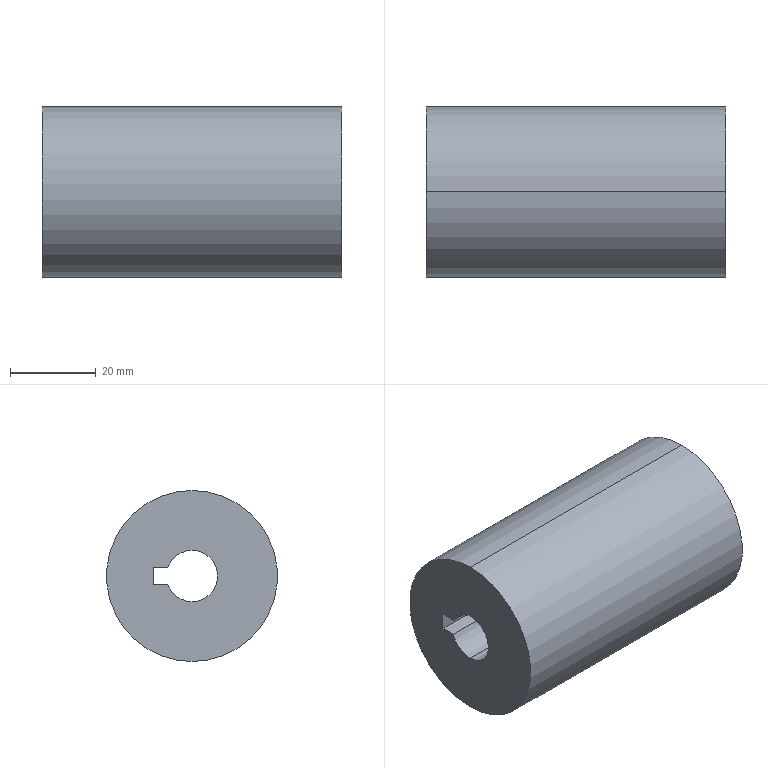Component | SolidWorks | Coupling2-1 | 1 solid | 10 faces | box 70 x 40 x 40 mm | volume 79176 mm3 | cylinder 5 | plane 5 | commonest cylinder face diameters 12 x3 40 x2
build123d program:
from build123d import *

# Parameters (mm, degrees)
SKETCH1_R      = 20
EXTRUDE1_DEPTH = 70


with BuildPart() as part:
    # Sketch1 → Extrude1 (new body)
    with BuildSketch(Plane.XY):
        Circle(SKETCH1_R)
        with BuildLine():
            Line((-2, 9), (2, 9))
            Line((2, 9), (2, 5.657))
            ThreePointArc((2, 5.657), (0, -6), (-2, 5.657))
            Line((-2, 5.657), (-2, 9))
        make_face(mode=Mode.SUBTRACT)
    extrude(amount=EXTRUDE1_DEPTH)


solid = part.part

# Placed as in the assembly
solid = solid.moved(Location((-87.284, 175.983, 58.736), (0, 90, 0)))
STEP:
#1=CARTESIAN_POINT('',(-0.6805,6.928,2.549));
#2=VERTEX_POINT('',#1);
#3=CARTESIAN_POINT('',(-0.6805,6.928,2.076));
#4=VERTEX_POINT('',#3);
#5=CARTESIAN_POINT('',(-0.6805,6.928,2.312));
#6=DIRECTION('',(1.,0.,0.));
#7=DIRECTION('',(0.,0.,-1.));
#8=AXIS2_PLACEMENT_3D('',#5,#6,#7);
#9=CIRCLE('',#8,0.2362);
#10=EDGE_CURVE('',#2,#4,#9,.T.);
#11=ORIENTED_EDGE('',*,*,#10,.T.);
#12=CARTESIAN_POINT('',(-3.436,6.928,2.076));
#13=VERTEX_POINT('',#12);
#14=CARTESIAN_POINT('',(-0.6805,6.928,2.076));
#15=DIRECTION('',(-1.,-0.,-0.));
#16=VECTOR('',#15,39.37);
#17=LINE('',#14,#16);
#18=EDGE_CURVE('',#4,#13,#17,.T.);
#19=ORIENTED_EDGE('',*,*,#18,.T.);
#20=CARTESIAN_POINT('',(-3.436,6.928,2.549));
#21=VERTEX_POINT('',#20);
#22=CARTESIAN_POINT('',(-3.436,6.928,2.312));
#23=DIRECTION('',(1.,0.,0.));
#24=DIRECTION('',(0.,0.,-1.));
#25=AXIS2_PLACEMENT_3D('',#22,#23,#24);
#26=CIRCLE('',#25,0.2362);
#27=EDGE_CURVE('',#21,#13,#26,.T.);
#28=ORIENTED_EDGE('',*,*,#27,.F.);
#29=CARTESIAN_POINT('',(-0.6805,6.928,2.549));
#30=DIRECTION('',(-1.,-0.,-0.));
#31=VECTOR('',#30,39.37);
#32=LINE('',#29,#31);
#33=EDGE_CURVE('',#2,#21,#32,.T.);
#34=ORIENTED_EDGE('',*,*,#33,.F.);
#35=EDGE_LOOP('',(#11,#19,#28,#34));
#36=FACE_OUTER_BOUND('',#35,.T.);
#37=CARTESIAN_POINT('',(-0.6805,6.928,2.312));
#38=DIRECTION('',(-1.,-0.,-0.));
#39=DIRECTION('',(0.,0.,1.));
#40=AXIS2_PLACEMENT_3D('',#37,#38,#39);
#41=CYLINDRICAL_SURFACE('',#40,0.2362);
#42=ADVANCED_FACE('',(#36),#41,.F.);
#43=CARTESIAN_POINT('',(-0.6805,7.151,2.391));
#44=VERTEX_POINT('',#43);
#45=CARTESIAN_POINT('',(-0.6805,6.928,2.312));
#46=DIRECTION('',(1.,0.,0.));
#47=DIRECTION('',(0.,0.,-1.));
#48=AXIS2_PLACEMENT_3D('',#45,#46,#47);
#49=CIRCLE('',#48,0.2362);
#50=EDGE_CURVE('',#44,#2,#49,.T.);
#51=ORIENTED_EDGE('',*,*,#50,.T.);
#52=ORIENTED_EDGE('',*,*,#33,.T.);
#53=CARTESIAN_POINT('',(-3.436,7.151,2.391));
#54=VERTEX_POINT('',#53);
#55=CARTESIAN_POINT('',(-3.436,6.928,2.312));
#56=DIRECTION('',(1.,0.,0.));
#57=DIRECTION('',(0.,0.,-1.));
#58=AXIS2_PLACEMENT_3D('',#55,#56,#57);
#59=CIRCLE('',#58,0.2362);
#60=EDGE_CURVE('',#54,#21,#59,.T.);
#61=ORIENTED_EDGE('',*,*,#60,.F.);
#62=CARTESIAN_POINT('',(-0.6805,7.151,2.391));
#63=DIRECTION('',(-1.,-0.,-0.));
#64=VECTOR('',#63,39.37);
#65=LINE('',#62,#64);
#66=EDGE_CURVE('',#44,#54,#65,.T.);
#67=ORIENTED_EDGE('',*,*,#66,.F.);
#68=EDGE_LOOP('',(#51,#52,#61,#67));
#69=FACE_OUTER_BOUND('',#68,.T.);
#70=CARTESIAN_POINT('',(-0.6805,6.928,2.312));
#71=DIRECTION('',(-1.,-0.,-0.));
#72=DIRECTION('',(0.,0.,1.));
#73=AXIS2_PLACEMENT_3D('',#70,#71,#72);
#74=CYLINDRICAL_SURFACE('',#73,0.2362);
#75=ADVANCED_FACE('',(#69),#74,.F.);
#76=CARTESIAN_POINT('',(-0.6805,6.928,1.525));
#77=VERTEX_POINT('',#76);
#78=CARTESIAN_POINT('',(-0.6805,6.928,3.1));
#79=VERTEX_POINT('',#78);
#80=CARTESIAN_POINT('',(-0.6805,6.928,2.312));
#81=DIRECTION('',(1.,0.,0.));
#82=DIRECTION('',(0.,0.,-1.));
#83=AXIS2_PLACEMENT_3D('',#80,#81,#82);
#84=CIRCLE('',#83,0.7874);
#85=EDGE_CURVE('',#77,#79,#84,.T.);
#86=ORIENTED_EDGE('',*,*,#85,.F.);
#87=CARTESIAN_POINT('',(-3.436,6.928,1.525));
#88=VERTEX_POINT('',#87);
#89=CARTESIAN_POINT('',(-0.6805,6.928,1.525));
#90=DIRECTION('',(-1.,-0.,-0.));
#91=VECTOR('',#90,39.37);
#92=LINE('',#89,#91);
#93=EDGE_CURVE('',#77,#88,#92,.T.);
#94=ORIENTED_EDGE('',*,*,#93,.T.);
#95=CARTESIAN_POINT('',(-3.436,6.928,3.1));
#96=VERTEX_POINT('',#95);
#97=CARTESIAN_POINT('',(-3.436,6.928,2.312));
#98=DIRECTION('',(1.,0.,0.));
#99=DIRECTION('',(0.,0.,-1.));
#100=AXIS2_PLACEMENT_3D('',#97,#98,#99);
#101=CIRCLE('',#100,0.7874);
#102=EDGE_CURVE('',#88,#96,#101,.T.);
#103=ORIENTED_EDGE('',*,*,#102,.T.);
#104=CARTESIAN_POINT('',(-0.6805,6.928,3.1));
#105=DIRECTION('',(-1.,-0.,-0.));
#106=VECTOR('',#105,39.37);
#107=LINE('',#104,#106);
#108=EDGE_CURVE('',#79,#96,#107,.T.);
#109=ORIENTED_EDGE('',*,*,#108,.F.);
#110=EDGE_LOOP('',(#86,#94,#103,#109));
#111=FACE_OUTER_BOUND('',#110,.T.);
#112=CARTESIAN_POINT('',(-0.6805,6.928,2.312));
#113=DIRECTION('',(-1.,-0.,-0.));
#114=DIRECTION('',(0.,0.,1.));
#115=AXIS2_PLACEMENT_3D('',#112,#113,#114);
#116=CYLINDRICAL_SURFACE('',#115,0.7874);
#117=ADVANCED_FACE('',(#111),#116,.T.);
#118=CARTESIAN_POINT('',(-0.6805,6.928,2.312));
#119=DIRECTION('',(1.,0.,0.));
#120=DIRECTION('',(0.,0.,-1.));
#121=AXIS2_PLACEMENT_3D('',#118,#119,#120);
#122=CIRCLE('',#121,0.7874);
#123=EDGE_CURVE('',#79,#77,#122,.T.);
#124=ORIENTED_EDGE('',*,*,#123,.T.);
#125=ORIENTED_EDGE('',*,*,#85,.T.);
#126=EDGE_LOOP('',(#124,#125));
#127=FACE_OUTER_BOUND('',#126,.T.);
#128=ORIENTED_EDGE('',*,*,#50,.F.);
#129=CARTESIAN_POINT('',(-0.6805,7.283,2.391));
#130=VERTEX_POINT('',#129);
#131=CARTESIAN_POINT('',(-0.6805,7.283,2.391));
#132=DIRECTION('',(0.,-1.,0.));
#133=VECTOR('',#132,39.37);
#134=LINE('',#131,#133);
#135=EDGE_CURVE('',#130,#44,#134,.T.);
#136=ORIENTED_EDGE('',*,*,#135,.F.);
#137=CARTESIAN_POINT('',(-0.6805,7.283,2.234));
#138=VERTEX_POINT('',#137);
#139=CARTESIAN_POINT('',(-0.6805,7.283,2.391));
#140=DIRECTION('',(-0.,0.,1.));
#141=VECTOR('',#140,39.37);
#142=LINE('',#139,#141);
#143=EDGE_CURVE('',#138,#130,#142,.T.);
#144=ORIENTED_EDGE('',*,*,#143,.F.);
#145=CARTESIAN_POINT('',(-0.6805,7.151,2.234));
#146=VERTEX_POINT('',#145);
#147=CARTESIAN_POINT('',(-0.6805,7.283,2.234));
#148=DIRECTION('',(-0.,1.,-0.));
#149=VECTOR('',#148,39.37);
#150=LINE('',#147,#149);
#151=EDGE_CURVE('',#146,#138,#150,.T.);
#152=ORIENTED_EDGE('',*,*,#151,.F.);
#153=CARTESIAN_POINT('',(-0.6805,6.928,2.312));
#154=DIRECTION('',(1.,0.,0.));
#155=DIRECTION('',(0.,0.,-1.));
#156=AXIS2_PLACEMENT_3D('',#153,#154,#155);
#157=CIRCLE('',#156,0.2362);
#158=EDGE_CURVE('',#4,#146,#157,.T.);
#159=ORIENTED_EDGE('',*,*,#158,.F.);
#160=ORIENTED_EDGE('',*,*,#10,.F.);
#161=EDGE_LOOP('',(#128,#136,#144,#152,#159,#160));
#162=FACE_BOUND('',#161,.T.);
#163=CARTESIAN_POINT('',(-0.6805,6.928,2.312));
#164=DIRECTION('',(1.,0.,0.));
#165=DIRECTION('',(0.,-0.,-1.));
#166=AXIS2_PLACEMENT_3D('',#163,#164,#165);
#167=PLANE('',#166);
#168=ADVANCED_FACE('',(#127,#162),#167,.T.);
#169=CARTESIAN_POINT('',(-3.436,6.928,2.312));
#170=DIRECTION('',(1.,0.,0.));
#171=DIRECTION('',(0.,0.,-1.));
#172=AXIS2_PLACEMENT_3D('',#169,#170,#171);
#173=CIRCLE('',#172,0.7874);
#174=EDGE_CURVE('',#96,#88,#173,.T.);
#175=ORIENTED_EDGE('',*,*,#174,.F.);
#176=ORIENTED_EDGE('',*,*,#102,.F.);
#177=EDGE_LOOP('',(#175,#176));
#178=FACE_OUTER_BOUND('',#177,.T.);
#179=CARTESIAN_POINT('',(-3.436,7.283,2.391));
#180=VERTEX_POINT('',#179);
#181=CARTESIAN_POINT('',(-3.436,7.283,2.391));
#182=DIRECTION('',(0.,-1.,0.));
#183=VECTOR('',#182,39.37);
#184=LINE('',#181,#183);
#185=EDGE_CURVE('',#180,#54,#184,.T.);
#186=ORIENTED_EDGE('',*,*,#185,.T.);
#187=ORIENTED_EDGE('',*,*,#60,.T.);
#188=ORIENTED_EDGE('',*,*,#27,.T.);
#189=CARTESIAN_POINT('',(-3.436,7.151,2.234));
#190=VERTEX_POINT('',#189);
#191=CARTESIAN_POINT('',(-3.436,6.928,2.312));
#192=DIRECTION('',(1.,0.,0.));
#193=DIRECTION('',(0.,0.,-1.));
#194=AXIS2_PLACEMENT_3D('',#191,#192,#193);
#195=CIRCLE('',#194,0.2362);
#196=EDGE_CURVE('',#13,#190,#195,.T.);
#197=ORIENTED_EDGE('',*,*,#196,.T.);
#198=CARTESIAN_POINT('',(-3.436,7.283,2.234));
#199=VERTEX_POINT('',#198);
#200=CARTESIAN_POINT('',(-3.436,7.283,2.234));
#201=DIRECTION('',(-0.,1.,-0.));
#202=VECTOR('',#201,39.37);
#203=LINE('',#200,#202);
#204=EDGE_CURVE('',#190,#199,#203,.T.);
#205=ORIENTED_EDGE('',*,*,#204,.T.);
#206=CARTESIAN_POINT('',(-3.436,7.283,2.391));
#207=DIRECTION('',(-0.,0.,1.));
#208=VECTOR('',#207,39.37);
#209=LINE('',#206,#208);
#210=EDGE_CURVE('',#199,#180,#209,.T.);
#211=ORIENTED_EDGE('',*,*,#210,.T.);
#212=EDGE_LOOP('',(#186,#187,#188,#197,#205,#211));
#213=FACE_BOUND('',#212,.T.);
#214=CARTESIAN_POINT('',(-3.436,6.928,2.312));
#215=DIRECTION('',(1.,0.,0.));
#216=DIRECTION('',(0.,-0.,-1.));
#217=AXIS2_PLACEMENT_3D('',#214,#215,#216);
#218=PLANE('',#217);
#219=ADVANCED_FACE('',(#178,#213),#218,.F.);
#220=ORIENTED_EDGE('',*,*,#93,.F.);
#221=ORIENTED_EDGE('',*,*,#123,.F.);
#222=ORIENTED_EDGE('',*,*,#108,.T.);
#223=ORIENTED_EDGE('',*,*,#174,.T.);
#224=EDGE_LOOP('',(#220,#221,#222,#223));
#225=FACE_OUTER_BOUND('',#224,.T.);
#226=CARTESIAN_POINT('',(-0.6805,6.928,2.312));
#227=DIRECTION('',(-1.,-0.,-0.));
#228=DIRECTION('',(0.,0.,1.));
#229=AXIS2_PLACEMENT_3D('',#226,#227,#228);
#230=CYLINDRICAL_SURFACE('',#229,0.7874);
#231=ADVANCED_FACE('',(#225),#230,.T.);
#232=ORIENTED_EDGE('',*,*,#185,.F.);
#233=CARTESIAN_POINT('',(-0.6805,7.283,2.391));
#234=DIRECTION('',(-1.,-0.,-0.));
#235=VECTOR('',#234,39.37);
#236=LINE('',#233,#235);
#237=EDGE_CURVE('',#130,#180,#236,.T.);
#238=ORIENTED_EDGE('',*,*,#237,.F.);
#239=ORIENTED_EDGE('',*,*,#135,.T.);
#240=ORIENTED_EDGE('',*,*,#66,.T.);
#241=EDGE_LOOP('',(#232,#238,#239,#240));
#242=FACE_OUTER_BOUND('',#241,.T.);
#243=CARTESIAN_POINT('',(-0.6805,7.283,2.391));
#244=DIRECTION('',(0.,-0.,-1.));
#245=DIRECTION('',(-0.,1.,-0.));
#246=AXIS2_PLACEMENT_3D('',#243,#244,#245);
#247=PLANE('',#246);
#248=ADVANCED_FACE('',(#242),#247,.T.);
#249=ORIENTED_EDGE('',*,*,#18,.F.);
#250=ORIENTED_EDGE('',*,*,#158,.T.);
#251=CARTESIAN_POINT('',(-0.6805,7.151,2.234));
#252=DIRECTION('',(-1.,-0.,-0.));
#253=VECTOR('',#252,39.37);
#254=LINE('',#251,#253);
#255=EDGE_CURVE('',#146,#190,#254,.T.);
#256=ORIENTED_EDGE('',*,*,#255,.T.);
#257=ORIENTED_EDGE('',*,*,#196,.F.);
#258=EDGE_LOOP('',(#249,#250,#256,#257));
#259=FACE_OUTER_BOUND('',#258,.T.);
#260=CARTESIAN_POINT('',(-0.6805,6.928,2.312));
#261=DIRECTION('',(-1.,-0.,-0.));
#262=DIRECTION('',(0.,0.,1.));
#263=AXIS2_PLACEMENT_3D('',#260,#261,#262);
#264=CYLINDRICAL_SURFACE('',#263,0.2362);
#265=ADVANCED_FACE('',(#259),#264,.F.);
#266=ORIENTED_EDGE('',*,*,#204,.F.);
#267=ORIENTED_EDGE('',*,*,#255,.F.);
#268=ORIENTED_EDGE('',*,*,#151,.T.);
#269=CARTESIAN_POINT('',(-0.6805,7.283,2.234));
#270=DIRECTION('',(-1.,-0.,-0.));
#271=VECTOR('',#270,39.37);
#272=LINE('',#269,#271);
#273=EDGE_CURVE('',#138,#199,#272,.T.);
#274=ORIENTED_EDGE('',*,*,#273,.T.);
#275=EDGE_LOOP('',(#266,#267,#268,#274));
#276=FACE_OUTER_BOUND('',#275,.T.);
#277=CARTESIAN_POINT('',(-0.6805,7.283,2.234));
#278=DIRECTION('',(-0.,0.,1.));
#279=DIRECTION('',(0.,-1.,0.));
#280=AXIS2_PLACEMENT_3D('',#277,#278,#279);
#281=PLANE('',#280);
#282=ADVANCED_FACE('',(#276),#281,.T.);
#283=ORIENTED_EDGE('',*,*,#210,.F.);
#284=ORIENTED_EDGE('',*,*,#273,.F.);
#285=ORIENTED_EDGE('',*,*,#143,.T.);
#286=ORIENTED_EDGE('',*,*,#237,.T.);
#287=EDGE_LOOP('',(#283,#284,#285,#286));
#288=FACE_OUTER_BOUND('',#287,.T.);
#289=CARTESIAN_POINT('',(-0.6805,7.283,2.391));
#290=DIRECTION('',(0.,-1.,0.));
#291=DIRECTION('',(-1.,-0.,-0.));
#292=AXIS2_PLACEMENT_3D('',#289,#290,#291);
#293=PLANE('',#292);
#294=ADVANCED_FACE('',(#288),#293,.T.);
#295=CLOSED_SHELL('',(#42,#75,#117,#168,#219,#231,#248,#265,#282,#294));
#296=MANIFOLD_SOLID_BREP('',#295);
#297=CARTESIAN_POINT('',(0.,0.,0.));
#298=DIRECTION('',(0.,0.,1.));
#299=DIRECTION('',(1.,0.,0.));
#300=AXIS2_PLACEMENT_3D('',#297,#298,#299);
#301=(LENGTH_UNIT()NAMED_UNIT(*)SI_UNIT($,.METRE.));
#302=LENGTH_MEASURE_WITH_UNIT(LENGTH_MEASURE(0.0254),#301);
#303=DIMENSIONAL_EXPONENTS(1.,0.,0.,0.,0.,0.,0.);
#304=(CONVERSION_BASED_UNIT('',#302)LENGTH_UNIT()NAMED_UNIT(#303));
#305=UNCERTAINTY_MEASURE_WITH_UNIT(LENGTH_MEASURE(0.00001),#304,'','');
#306=(NAMED_UNIT(*)PLANE_ANGLE_UNIT()SI_UNIT($,.RADIAN.));
#307=(NAMED_UNIT(*)SI_UNIT($,.STERADIAN.)SOLID_ANGLE_UNIT());
#308=(GEOMETRIC_REPRESENTATION_CONTEXT(3)GLOBAL_UNCERTAINTY_ASSIGNED_CONTEXT((#305))GLOBAL_UNIT_ASSIGNED_CONTEXT((#304,#306,#307))REPRESENTATION_CONTEXT('',''));
#309=ADVANCED_BREP_SHAPE_REPRESENTATION('',(#296,#300),#308);
#310=COLOUR_RGB('',0.7922,0.8196,0.9333);
#311=FILL_AREA_STYLE_COLOUR('',#310);
#312=FILL_AREA_STYLE('',(#311));
#313=SURFACE_STYLE_FILL_AREA(#312);
#314=SURFACE_SIDE_STYLE('',(#313));
#315=SURFACE_STYLE_USAGE(.BOTH.,#314);
#316=PRESENTATION_STYLE_ASSIGNMENT((#315));
#317=STYLED_ITEM('',(#316),#296);
#318=(LENGTH_UNIT()NAMED_UNIT(*)SI_UNIT($,.METRE.));
#319=LENGTH_MEASURE_WITH_UNIT(LENGTH_MEASURE(0.0254),#318);
#320=DIMENSIONAL_EXPONENTS(1.,0.,0.,0.,0.,0.,0.);
#321=(CONVERSION_BASED_UNIT('',#319)LENGTH_UNIT()NAMED_UNIT(#320));
#322=UNCERTAINTY_MEASURE_WITH_UNIT(LENGTH_MEASURE(0.00001),#321,'','');
#323=(NAMED_UNIT(*)PLANE_ANGLE_UNIT()SI_UNIT($,.RADIAN.));
#324=(NAMED_UNIT(*)SI_UNIT($,.STERADIAN.)SOLID_ANGLE_UNIT());
#325=(GEOMETRIC_REPRESENTATION_CONTEXT(3)GLOBAL_UNCERTAINTY_ASSIGNED_CONTEXT((#322))GLOBAL_UNIT_ASSIGNED_CONTEXT((#321,#323,#324))REPRESENTATION_CONTEXT('',''));
#326=MECHANICAL_DESIGN_GEOMETRIC_PRESENTATION_REPRESENTATION('',(#317),#325);
#327=PRESENTATION_LAYER_ASSIGNMENT('','',(#317));